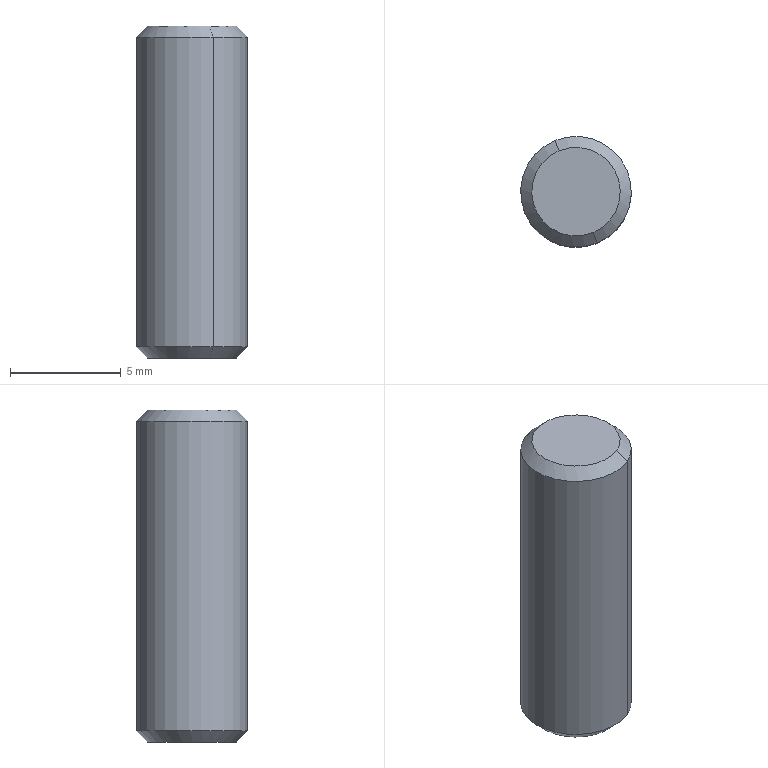Component | SolidWorks | DowelPin5X15L-3 | 1 solid | 8 faces | box 5 x 5 x 15 mm | volume 291 mm3 | cone 4 | cylinder 2 | plane 2 | commonest cylinder face diameters 5 x2
build123d program:
from build123d import *

# Parameters (mm, degrees)
SKETCH1_R           = 2.5
BOSS_EXTRUDE1_DEPTH = 15
CHAMFER1_SIZE       = 0.5


with BuildPart() as part:
    # Sketch1 → Boss-Extrude1 (new body)
    with BuildSketch(Plane(origin=(0, 0, 0), x_dir=(1, 0, 0), z_dir=(0, 1, 0))):
        with Locations(Location((0, 0, 0), (0, 0, 270))):
            Circle(SKETCH1_R)
    extrude(amount=BOSS_EXTRUDE1_DEPTH)

    # Chamfer1
    chamfer1_edges = [part.edges().sort_by_distance(p)[0] for p in [
        (0, 0, -2.5),
        (0, 15, -2.5),
    ]]
    chamfer(chamfer1_edges, length=CHAMFER1_SIZE)


solid = part.part

# Placed as in the assembly
solid = solid.moved(Location((5.932, -7.687, 380.197), (90, 0, 0)))
STEP:
#1=CARTESIAN_POINT('',(0.2637,-0.3754,14.968));
#2=VERTEX_POINT('',#1);
#3=CARTESIAN_POINT('',(0.2034,-0.2299,14.968));
#4=VERTEX_POINT('',#3);
#5=CARTESIAN_POINT('',(0.2335,-0.3026,14.968));
#6=DIRECTION('',(0.,0.,-1.));
#7=DIRECTION('',(-0.383,0.9237,0.));
#8=AXIS2_PLACEMENT_3D('',#5,#6,#7);
#9=CIRCLE('',#8,0.07874);
#10=EDGE_CURVE('',#2,#4,#9,.T.);
#11=ORIENTED_EDGE('',*,*,#10,.F.);
#12=CARTESIAN_POINT('',(0.2712,-0.3936,14.988));
#13=VERTEX_POINT('',#12);
#14=CARTESIAN_POINT('',(0.2712,-0.3936,14.988));
#15=DIRECTION('',(0.2709,-0.6532,0.7071));
#16=VECTOR('',#15,39.37);
#17=LINE('',#14,#16);
#18=EDGE_CURVE('',#2,#13,#17,.T.);
#19=ORIENTED_EDGE('',*,*,#18,.T.);
#20=CARTESIAN_POINT('',(0.1958,-0.2117,14.988));
#21=VERTEX_POINT('',#20);
#22=CARTESIAN_POINT('',(0.2335,-0.3026,14.988));
#23=DIRECTION('',(-0.,-0.,1.));
#24=DIRECTION('',(-0.383,0.9237,0.));
#25=AXIS2_PLACEMENT_3D('',#22,#23,#24);
#26=CIRCLE('',#25,0.09843);
#27=EDGE_CURVE('',#21,#13,#26,.T.);
#28=ORIENTED_EDGE('',*,*,#27,.F.);
#29=CARTESIAN_POINT('',(0.1958,-0.2117,14.988));
#30=DIRECTION('',(-0.2709,0.6532,0.7071));
#31=VECTOR('',#30,39.37);
#32=LINE('',#29,#31);
#33=EDGE_CURVE('',#4,#21,#32,.T.);
#34=ORIENTED_EDGE('',*,*,#33,.F.);
#35=EDGE_LOOP('',(#11,#19,#28,#34));
#36=FACE_OUTER_BOUND('',#35,.T.);
#37=CARTESIAN_POINT('',(0.2335,-0.3026,14.988));
#38=DIRECTION('',(-0.,-0.,1.));
#39=DIRECTION('',(-0.383,0.9237,0.));
#40=AXIS2_PLACEMENT_3D('',#37,#38,#39);
#41=CONICAL_SURFACE('',#40,0.09843,0.7854);
#42=ADVANCED_FACE('',(#36),#41,.T.);
#43=CARTESIAN_POINT('',(0.2034,-0.2299,15.559));
#44=VERTEX_POINT('',#43);
#45=CARTESIAN_POINT('',(0.2637,-0.3754,15.559));
#46=VERTEX_POINT('',#45);
#47=CARTESIAN_POINT('',(0.2335,-0.3026,15.559));
#48=DIRECTION('',(-0.,-0.,1.));
#49=DIRECTION('',(-0.383,0.9237,0.));
#50=AXIS2_PLACEMENT_3D('',#47,#48,#49);
#51=CIRCLE('',#50,0.07874);
#52=EDGE_CURVE('',#44,#46,#51,.T.);
#53=ORIENTED_EDGE('',*,*,#52,.F.);
#54=CARTESIAN_POINT('',(0.1958,-0.2117,15.539));
#55=VERTEX_POINT('',#54);
#56=CARTESIAN_POINT('',(0.2034,-0.2299,15.559));
#57=DIRECTION('',(-0.2709,0.6532,-0.7071));
#58=VECTOR('',#57,39.37);
#59=LINE('',#56,#58);
#60=EDGE_CURVE('',#44,#55,#59,.T.);
#61=ORIENTED_EDGE('',*,*,#60,.T.);
#62=CARTESIAN_POINT('',(0.2712,-0.3936,15.539));
#63=VERTEX_POINT('',#62);
#64=CARTESIAN_POINT('',(0.2335,-0.3026,15.539));
#65=DIRECTION('',(0.,0.,-1.));
#66=DIRECTION('',(-0.383,0.9237,0.));
#67=AXIS2_PLACEMENT_3D('',#64,#65,#66);
#68=CIRCLE('',#67,0.09843);
#69=EDGE_CURVE('',#63,#55,#68,.T.);
#70=ORIENTED_EDGE('',*,*,#69,.F.);
#71=CARTESIAN_POINT('',(0.2637,-0.3754,15.559));
#72=DIRECTION('',(0.2709,-0.6532,-0.7071));
#73=VECTOR('',#72,39.37);
#74=LINE('',#71,#73);
#75=EDGE_CURVE('',#46,#63,#74,.T.);
#76=ORIENTED_EDGE('',*,*,#75,.F.);
#77=EDGE_LOOP('',(#53,#61,#70,#76));
#78=FACE_OUTER_BOUND('',#77,.T.);
#79=CARTESIAN_POINT('',(0.2335,-0.3026,15.559));
#80=DIRECTION('',(0.,0.,-1.));
#81=DIRECTION('',(0.383,-0.9237,0.));
#82=AXIS2_PLACEMENT_3D('',#79,#80,#81);
#83=CONICAL_SURFACE('',#82,0.07874,0.7854);
#84=ADVANCED_FACE('',(#78),#83,.T.);
#85=ORIENTED_EDGE('',*,*,#69,.T.);
#86=CARTESIAN_POINT('',(0.1958,-0.2117,15.559));
#87=DIRECTION('',(0.,0.,-1.));
#88=VECTOR('',#87,39.37);
#89=LINE('',#86,#88);
#90=EDGE_CURVE('',#55,#21,#89,.T.);
#91=ORIENTED_EDGE('',*,*,#90,.T.);
#92=ORIENTED_EDGE('',*,*,#27,.T.);
#93=CARTESIAN_POINT('',(0.2712,-0.3936,15.559));
#94=DIRECTION('',(0.,0.,-1.));
#95=VECTOR('',#94,39.37);
#96=LINE('',#93,#95);
#97=EDGE_CURVE('',#63,#13,#96,.T.);
#98=ORIENTED_EDGE('',*,*,#97,.F.);
#99=EDGE_LOOP('',(#85,#91,#92,#98));
#100=FACE_OUTER_BOUND('',#99,.T.);
#101=CARTESIAN_POINT('',(0.2335,-0.3026,15.559));
#102=DIRECTION('',(0.,0.,-1.));
#103=DIRECTION('',(0.383,-0.9237,0.));
#104=AXIS2_PLACEMENT_3D('',#101,#102,#103);
#105=CYLINDRICAL_SURFACE('',#104,0.09843);
#106=ADVANCED_FACE('',(#100),#105,.T.);
#107=ORIENTED_EDGE('',*,*,#90,.F.);
#108=CARTESIAN_POINT('',(0.2335,-0.3026,15.539));
#109=DIRECTION('',(0.,0.,-1.));
#110=DIRECTION('',(-0.383,0.9237,0.));
#111=AXIS2_PLACEMENT_3D('',#108,#109,#110);
#112=CIRCLE('',#111,0.09843);
#113=EDGE_CURVE('',#55,#63,#112,.T.);
#114=ORIENTED_EDGE('',*,*,#113,.T.);
#115=ORIENTED_EDGE('',*,*,#97,.T.);
#116=CARTESIAN_POINT('',(0.2335,-0.3026,14.988));
#117=DIRECTION('',(-0.,-0.,1.));
#118=DIRECTION('',(-0.383,0.9237,0.));
#119=AXIS2_PLACEMENT_3D('',#116,#117,#118);
#120=CIRCLE('',#119,0.09843);
#121=EDGE_CURVE('',#13,#21,#120,.T.);
#122=ORIENTED_EDGE('',*,*,#121,.T.);
#123=EDGE_LOOP('',(#107,#114,#115,#122));
#124=FACE_OUTER_BOUND('',#123,.T.);
#125=CARTESIAN_POINT('',(0.2335,-0.3026,15.559));
#126=DIRECTION('',(0.,0.,-1.));
#127=DIRECTION('',(0.383,-0.9237,0.));
#128=AXIS2_PLACEMENT_3D('',#125,#126,#127);
#129=CYLINDRICAL_SURFACE('',#128,0.09843);
#130=ADVANCED_FACE('',(#124),#129,.T.);
#131=CARTESIAN_POINT('',(0.2335,-0.3026,15.559));
#132=DIRECTION('',(-0.,-0.,1.));
#133=DIRECTION('',(-0.383,0.9237,0.));
#134=AXIS2_PLACEMENT_3D('',#131,#132,#133);
#135=CIRCLE('',#134,0.07874);
#136=EDGE_CURVE('',#46,#44,#135,.T.);
#137=ORIENTED_EDGE('',*,*,#136,.T.);
#138=ORIENTED_EDGE('',*,*,#52,.T.);
#139=EDGE_LOOP('',(#137,#138));
#140=FACE_OUTER_BOUND('',#139,.T.);
#141=CARTESIAN_POINT('',(0.2335,-0.3026,15.559));
#142=DIRECTION('',(-0.,-0.,1.));
#143=DIRECTION('',(-0.383,0.9237,-0.));
#144=AXIS2_PLACEMENT_3D('',#141,#142,#143);
#145=PLANE('',#144);
#146=ADVANCED_FACE('',(#140),#145,.T.);
#147=CARTESIAN_POINT('',(0.2335,-0.3026,14.968));
#148=DIRECTION('',(0.,0.,-1.));
#149=DIRECTION('',(-0.383,0.9237,0.));
#150=AXIS2_PLACEMENT_3D('',#147,#148,#149);
#151=CIRCLE('',#150,0.07874);
#152=EDGE_CURVE('',#4,#2,#151,.T.);
#153=ORIENTED_EDGE('',*,*,#152,.T.);
#154=ORIENTED_EDGE('',*,*,#10,.T.);
#155=EDGE_LOOP('',(#153,#154));
#156=FACE_OUTER_BOUND('',#155,.T.);
#157=CARTESIAN_POINT('',(0.2335,-0.3026,14.968));
#158=DIRECTION('',(-0.,-0.,1.));
#159=DIRECTION('',(-0.383,0.9237,-0.));
#160=AXIS2_PLACEMENT_3D('',#157,#158,#159);
#161=PLANE('',#160);
#162=ADVANCED_FACE('',(#156),#161,.F.);
#163=ORIENTED_EDGE('',*,*,#60,.F.);
#164=ORIENTED_EDGE('',*,*,#136,.F.);
#165=ORIENTED_EDGE('',*,*,#75,.T.);
#166=ORIENTED_EDGE('',*,*,#113,.F.);
#167=EDGE_LOOP('',(#163,#164,#165,#166));
#168=FACE_OUTER_BOUND('',#167,.T.);
#169=CARTESIAN_POINT('',(0.2335,-0.3026,15.559));
#170=DIRECTION('',(0.,0.,-1.));
#171=DIRECTION('',(0.383,-0.9237,0.));
#172=AXIS2_PLACEMENT_3D('',#169,#170,#171);
#173=CONICAL_SURFACE('',#172,0.07874,0.7854);
#174=ADVANCED_FACE('',(#168),#173,.T.);
#175=ORIENTED_EDGE('',*,*,#18,.F.);
#176=ORIENTED_EDGE('',*,*,#152,.F.);
#177=ORIENTED_EDGE('',*,*,#33,.T.);
#178=ORIENTED_EDGE('',*,*,#121,.F.);
#179=EDGE_LOOP('',(#175,#176,#177,#178));
#180=FACE_OUTER_BOUND('',#179,.T.);
#181=CARTESIAN_POINT('',(0.2335,-0.3026,14.988));
#182=DIRECTION('',(-0.,-0.,1.));
#183=DIRECTION('',(-0.383,0.9237,0.));
#184=AXIS2_PLACEMENT_3D('',#181,#182,#183);
#185=CONICAL_SURFACE('',#184,0.09843,0.7854);
#186=ADVANCED_FACE('',(#180),#185,.T.);
#187=CLOSED_SHELL('',(#42,#84,#106,#130,#146,#162,#174,#186));
#188=MANIFOLD_SOLID_BREP('',#187);
#189=CARTESIAN_POINT('',(0.,0.,0.));
#190=DIRECTION('',(0.,0.,1.));
#191=DIRECTION('',(1.,0.,0.));
#192=AXIS2_PLACEMENT_3D('',#189,#190,#191);
#193=(LENGTH_UNIT()NAMED_UNIT(*)SI_UNIT($,.METRE.));
#194=LENGTH_MEASURE_WITH_UNIT(LENGTH_MEASURE(0.0254),#193);
#195=DIMENSIONAL_EXPONENTS(1.,0.,0.,0.,0.,0.,0.);
#196=(CONVERSION_BASED_UNIT('',#194)LENGTH_UNIT()NAMED_UNIT(#195));
#197=UNCERTAINTY_MEASURE_WITH_UNIT(LENGTH_MEASURE(0.00001),#196,'','');
#198=(NAMED_UNIT(*)PLANE_ANGLE_UNIT()SI_UNIT($,.RADIAN.));
#199=(NAMED_UNIT(*)SI_UNIT($,.STERADIAN.)SOLID_ANGLE_UNIT());
#200=(GEOMETRIC_REPRESENTATION_CONTEXT(3)GLOBAL_UNCERTAINTY_ASSIGNED_CONTEXT((#197))GLOBAL_UNIT_ASSIGNED_CONTEXT((#196,#198,#199))REPRESENTATION_CONTEXT('',''));
#201=ADVANCED_BREP_SHAPE_REPRESENTATION('',(#188,#192),#200);
#202=COLOUR_RGB('',0.7922,0.8196,0.9333);
#203=FILL_AREA_STYLE_COLOUR('',#202);
#204=FILL_AREA_STYLE('',(#203));
#205=SURFACE_STYLE_FILL_AREA(#204);
#206=SURFACE_SIDE_STYLE('',(#205));
#207=SURFACE_STYLE_USAGE(.BOTH.,#206);
#208=PRESENTATION_STYLE_ASSIGNMENT((#207));
#209=STYLED_ITEM('',(#208),#188);
#210=PRESENTATION_LAYER_ASSIGNMENT('','',(#209));
#211=(LENGTH_UNIT()NAMED_UNIT(*)SI_UNIT($,.METRE.));
#212=LENGTH_MEASURE_WITH_UNIT(LENGTH_MEASURE(0.0254),#211);
#213=DIMENSIONAL_EXPONENTS(1.,0.,0.,0.,0.,0.,0.);
#214=(CONVERSION_BASED_UNIT('',#212)LENGTH_UNIT()NAMED_UNIT(#213));
#215=UNCERTAINTY_MEASURE_WITH_UNIT(LENGTH_MEASURE(0.00001),#214,'','');
#216=(NAMED_UNIT(*)PLANE_ANGLE_UNIT()SI_UNIT($,.RADIAN.));
#217=(NAMED_UNIT(*)SI_UNIT($,.STERADIAN.)SOLID_ANGLE_UNIT());
#218=(GEOMETRIC_REPRESENTATION_CONTEXT(3)GLOBAL_UNCERTAINTY_ASSIGNED_CONTEXT((#215))GLOBAL_UNIT_ASSIGNED_CONTEXT((#214,#216,#217))REPRESENTATION_CONTEXT('',''));
#219=MECHANICAL_DESIGN_GEOMETRIC_PRESENTATION_REPRESENTATION('',(#209),#218);